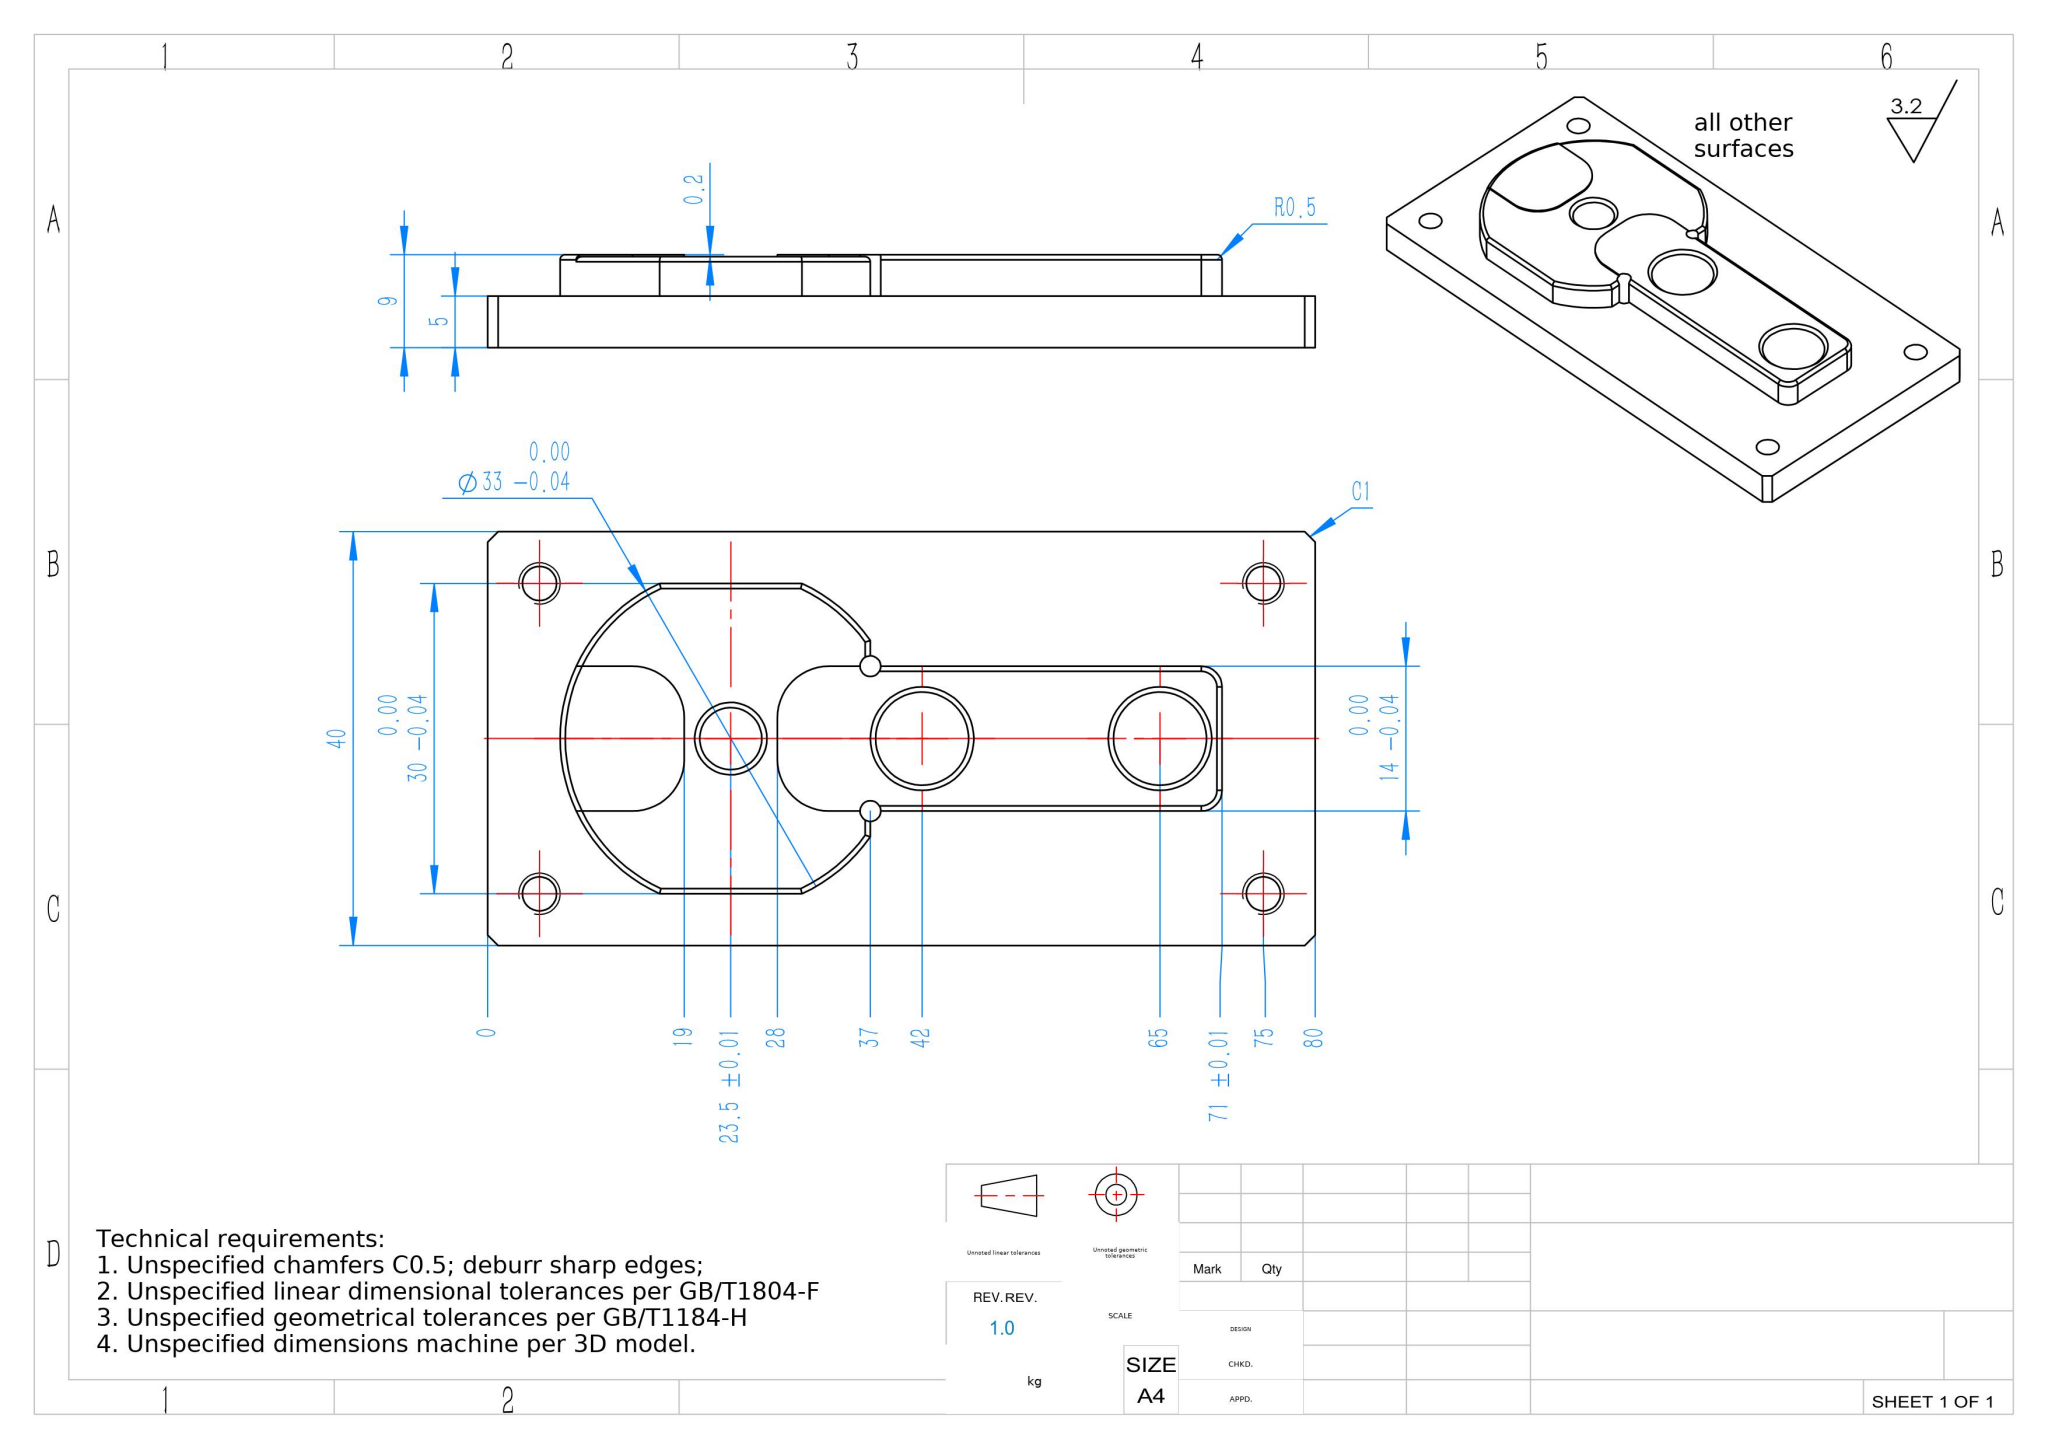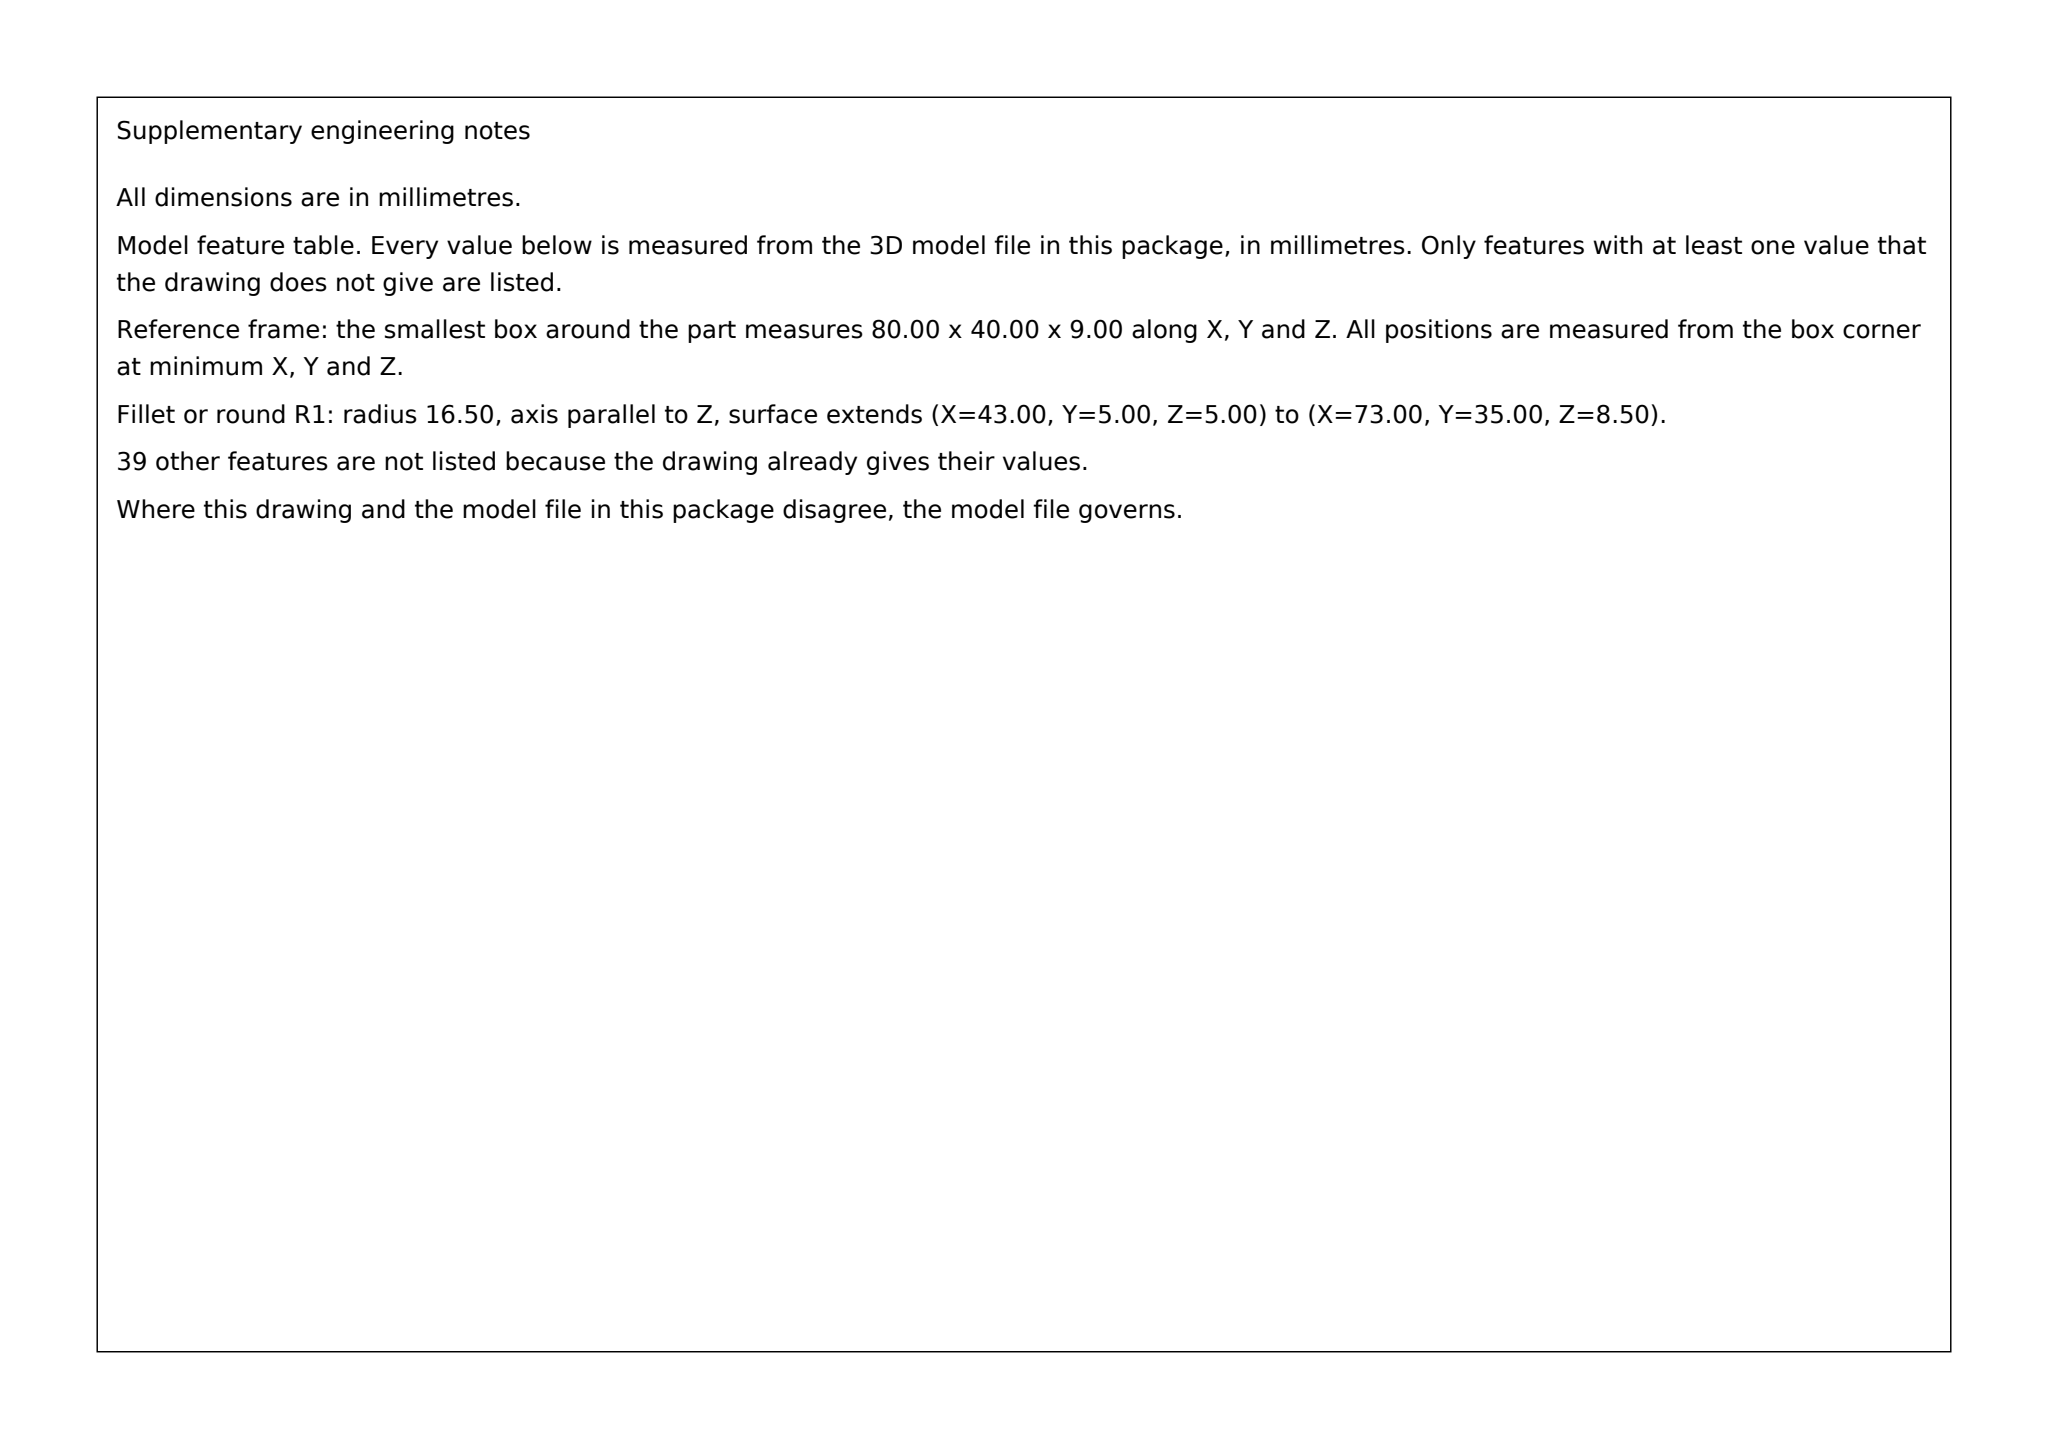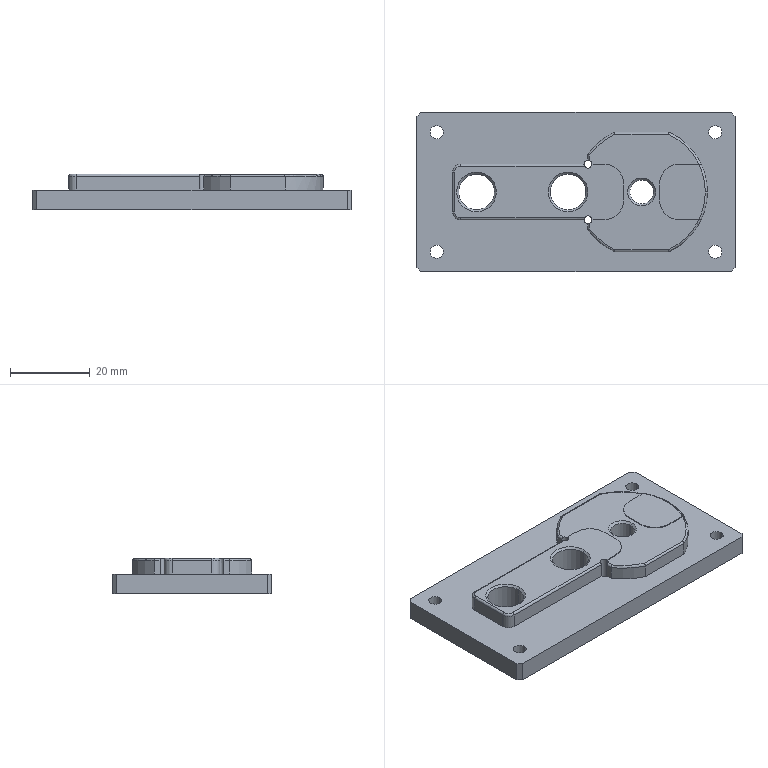Part | SolidWorks | mm | 1 solid | 80 faces | box 80 x 40 x 9 mm | volume 19295 mm3 | cylinder 34 | plane 26 | cone 12 | torus 8 | commonest cylinder face diameters 3.3 x8 1 x7 2 x4 9 x4 10 x4 33 x3 6 x2 4 x2